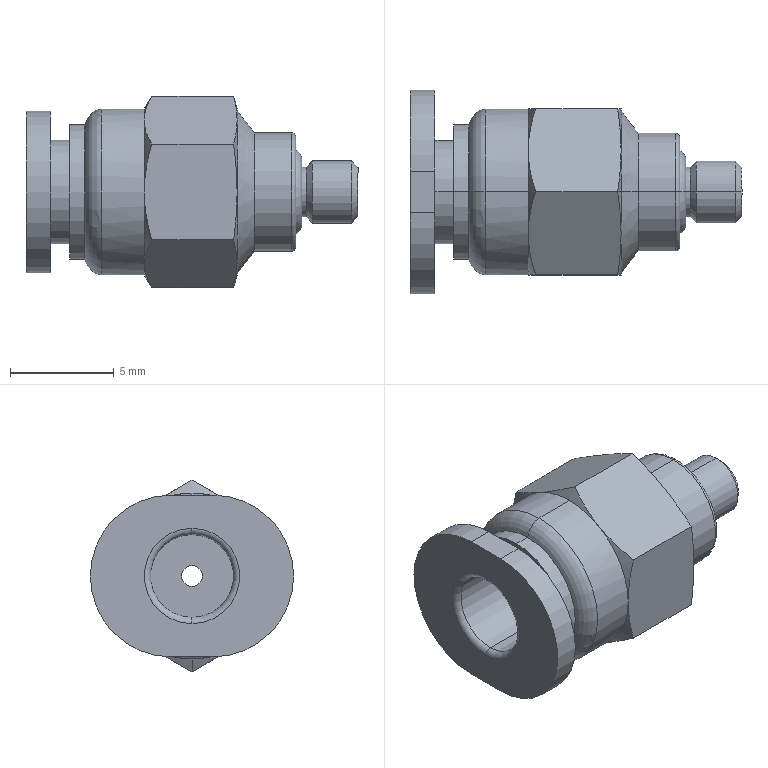Component | SolidWorks | WaterQuickConnector-10 | 1 solid | 62 faces | volume 456 mm3 | cylinder 20 | cone 19 | plane 15 | torus 8 | commonest cylinder face diameters 3 x2 1 x2 2.4 x2 4 x2 3.8 x2 5 x2 5.7 x2 6.5 x2